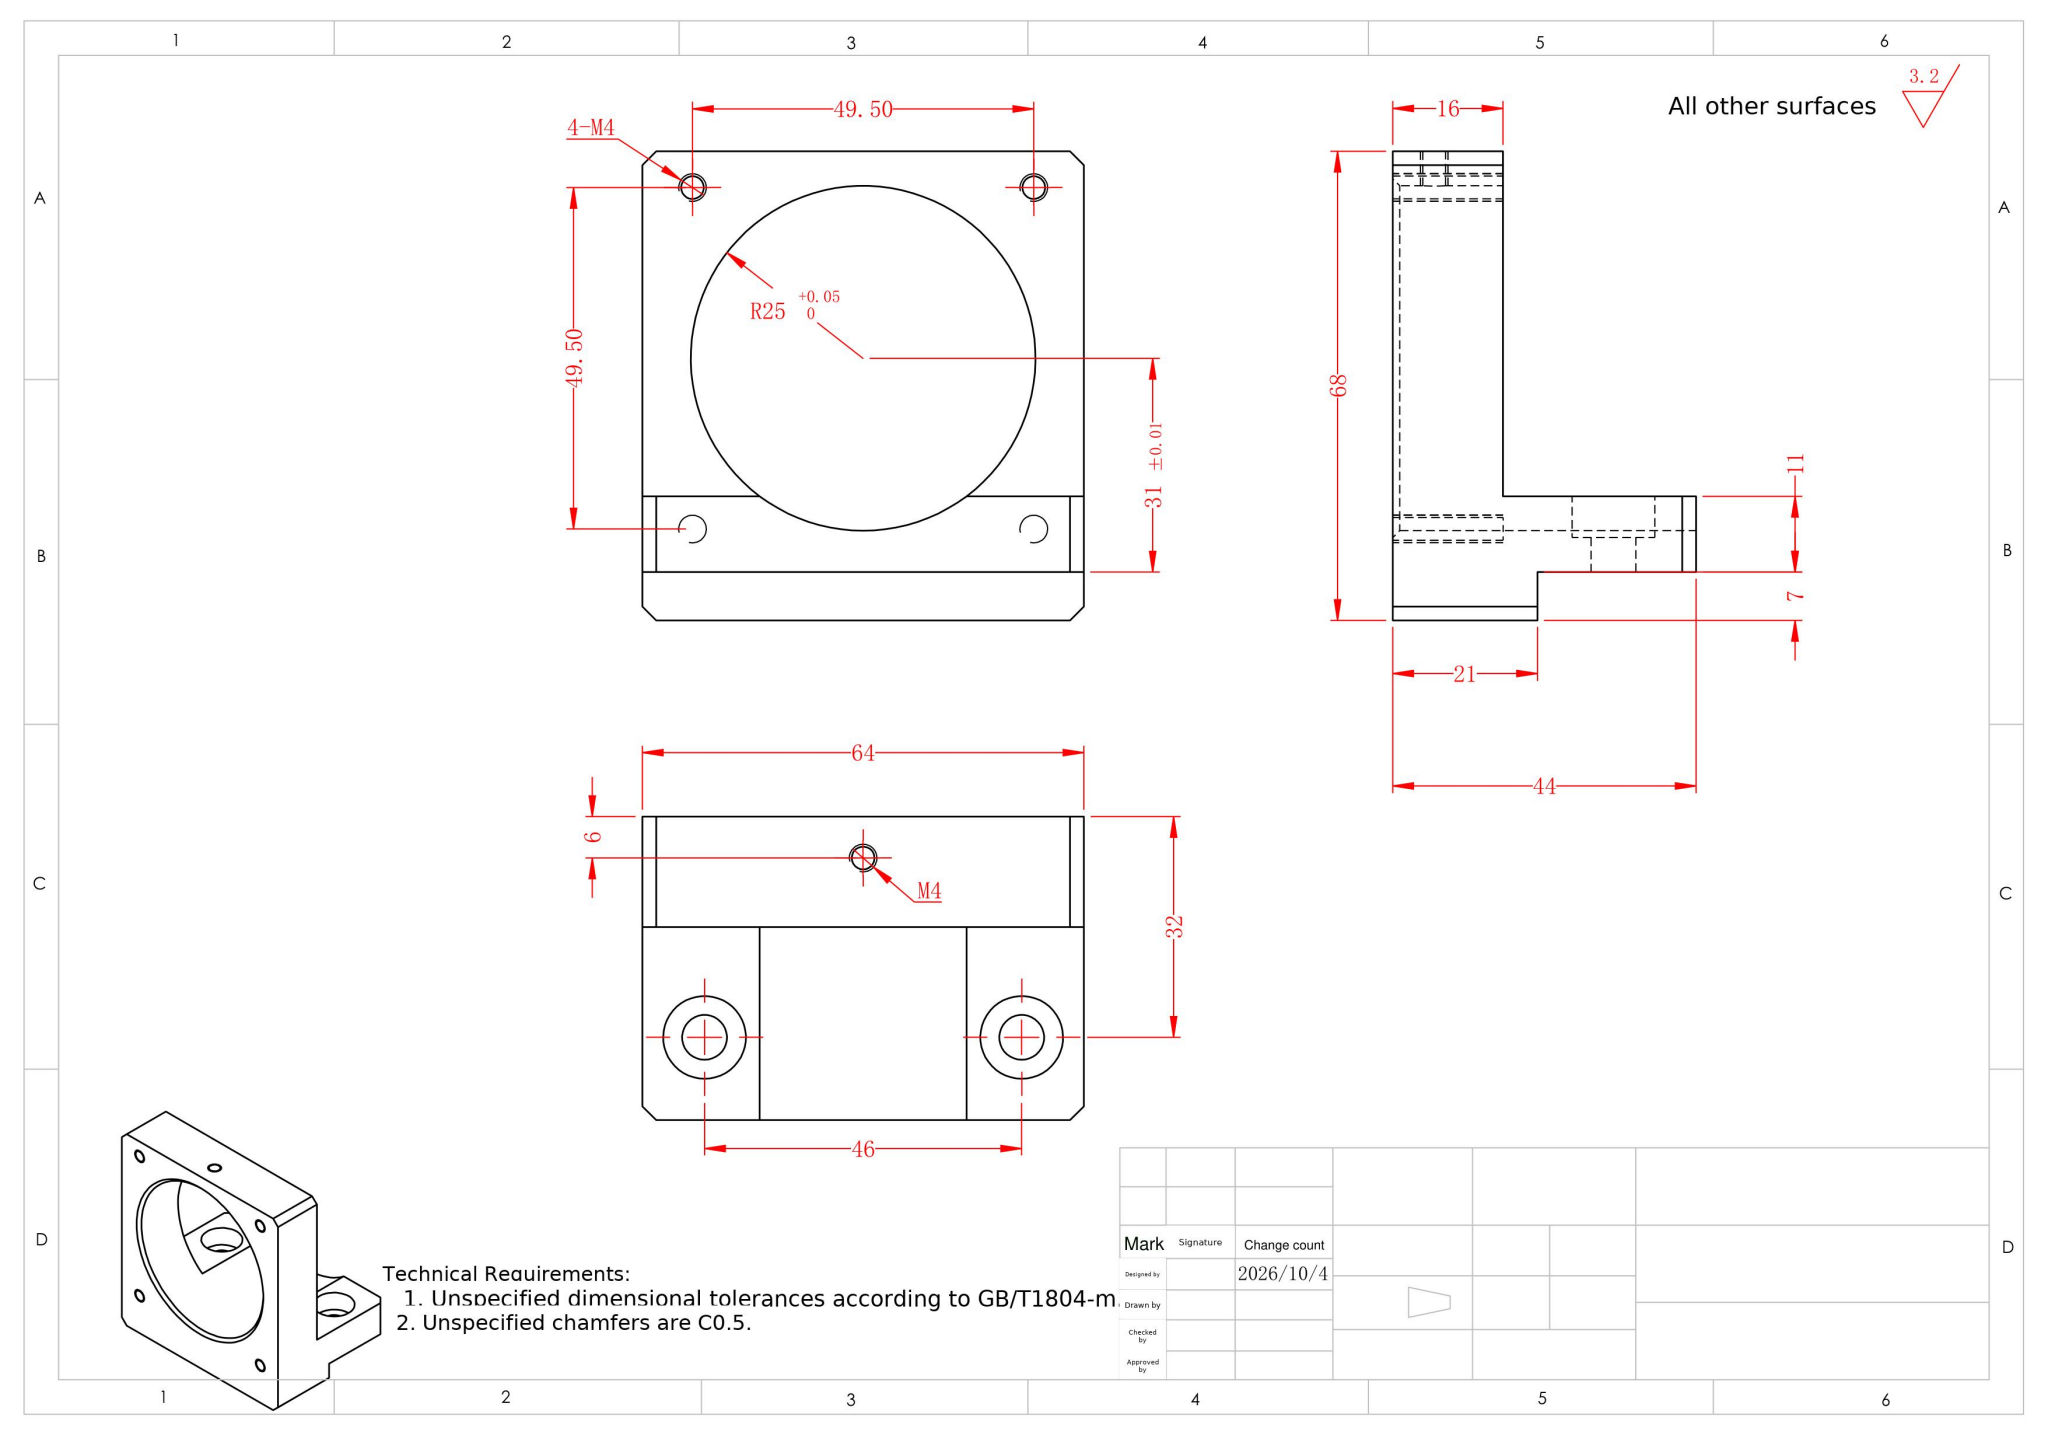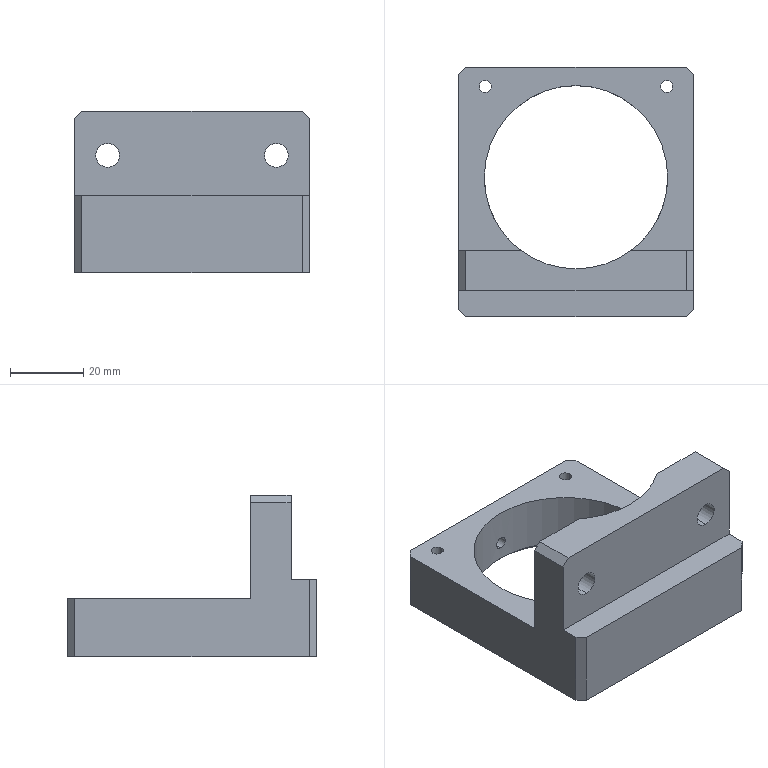Part | SolidWorks | mm | 1 solid | 43 faces | box 64 x 68 x 44 mm | volume 54756 mm3 | plane 21 | cylinder 20 | cone 2 | commonest cylinder face diameters 3.3 x10 12 x4 6.5 x4 50 x2
build123d program:
from build123d import *

# Parameters (mm, degrees)
SKETCH1_W                                       = 64
SKETCH1_H                                       = 68
SKETCH1_R                                       = 25
BOSS_EXTRUDE1_DEPTH                             = 16
M4_TAPPED_HOLE2_D                               = 3.3
M4_TAPPED_HOLE1_REACH                           = 87.871
M4_TAPPED_HOLE1_BORE_R                          = 1.65
CHAMFER2_SIZE                                   = 1
BOSS_EXTRUDE2_DEPTH                             = 28
M6_HEX_SOCKET_HEAD_CAP_SCREW_CBORE1_D           = 6.5
M6_HEX_SOCKET_HEAD_CAP_SCREW_CBORE1_CBORE_D     = 12
M6_HEX_SOCKET_HEAD_CAP_SCREW_CBORE1_CBORE_DEPTH = 6
SKETCH20_W                                      = 36.466
SKETCH20_H                                      = 26.571
CUT_EXTRUDE1_DEPTH                              = 110.683
CHAMFER3_SIZE                                   = 2


with BuildPart() as part:
    # Sketch1 → Boss-Extrude1 (new body)
    with BuildSketch(Plane.XY):
        with Locations((-17.938, 43.45)):
            Rectangle(SKETCH1_W, SKETCH1_H)
        with Locations((-17.938, 47.45)):
            Circle(SKETCH1_R, mode=Mode.SUBTRACT)
    extrude(amount=BOSS_EXTRUDE1_DEPTH)

    # M4 Tapped Hole2 (through all)
    with Locations(Plane(origin=(0, 0, 0), x_dir=(-1, 0, 0), z_dir=(0, 0, -1))):
        with Locations((-6.812, 72.2), (42.688, 72.2), (42.688, 22.7), (-6.812, 22.7)):
            Hole(M4_TAPPED_HOLE2_D / 2)

    # M4 Tapped Hole1 bore → M4 Tapped Hole1 (cut, up to next)
    with BuildSketch(Plane(origin=(0, 77.45, 0), x_dir=(1, 0, 0), z_dir=(0, 1, 0)), mode=Mode.PRIVATE) as m4_tapped_hole1_sk1:
        with Locations((-17.938, -6)):
            Circle(M4_TAPPED_HOLE1_BORE_R)
    m4_tapped_hole1_tool1 = extrude(m4_tapped_hole1_sk1.sketch, amount=-M4_TAPPED_HOLE1_REACH, mode=Mode.PRIVATE) & part.part
    add(m4_tapped_hole1_tool1.solids().sort_by_distance((-17.938, 77.45, 6))[0], mode=Mode.SUBTRACT)

    # Chamfer2
    chamfer2_edges = [part.edges().sort_by_distance(p)[0] for p in [
        (-42.938, 47.45, 0),
    ]]
    chamfer(chamfer2_edges, length=CHAMFER2_SIZE)

    # Sketch17 → Boss-Extrude2 (add)
    with BuildSketch(Plane.XY.offset(16)):
        with BuildLine():
            Line((-2.938, 27.45), (14.062, 27.45))
            Line((14.062, 27.45), (14.062, 9.45))
            Line((14.062, 9.45), (-49.938, 9.45))
            Line((-49.938, 9.45), (-49.938, 27.45))
            Line((-49.938, 27.45), (-32.938, 27.45))
            ThreePointArc((-32.938, 27.45), (-17.938, 22.45), (-2.938, 27.45))
        make_face()
    extrude(amount=BOSS_EXTRUDE2_DEPTH)

    # M6 Hex Socket Head Cap Screw CBORE1 (through all)
    with Locations(Plane(origin=(0, 27.45, 0), x_dir=(1, 0, 0), z_dir=(0, 1, 0))):
        with Locations((-40.938, -32), (5.062, -32)):
            CounterBoreHole(M6_HEX_SOCKET_HEAD_CAP_SCREW_CBORE1_D / 2, M6_HEX_SOCKET_HEAD_CAP_SCREW_CBORE1_CBORE_D / 2, M6_HEX_SOCKET_HEAD_CAP_SCREW_CBORE1_CBORE_DEPTH)

    # Sketch20 → Cut-Extrude1 (cut, through all)
    with BuildSketch(Plane.ZY.offset(49.938)):
        with Locations((39.233, 3.164)):
            Rectangle(SKETCH20_W, SKETCH20_H)
    extrude(amount=-CUT_EXTRUDE1_DEPTH, mode=Mode.SUBTRACT)

    # Chamfer3
    chamfer3_edges = [part.edges().sort_by_distance(p)[0] for p in [
        (-49.938, 21.95, 44),
        (-49.938, 77.45, 8),
        (14.062, 77.45, 8),
        (14.062, 21.95, 44),
        (14.062, 9.45, 10.5),
        (-49.938, 9.45, 10.5),
    ]]
    chamfer(chamfer3_edges, length=CHAMFER3_SIZE)


solid = part.part